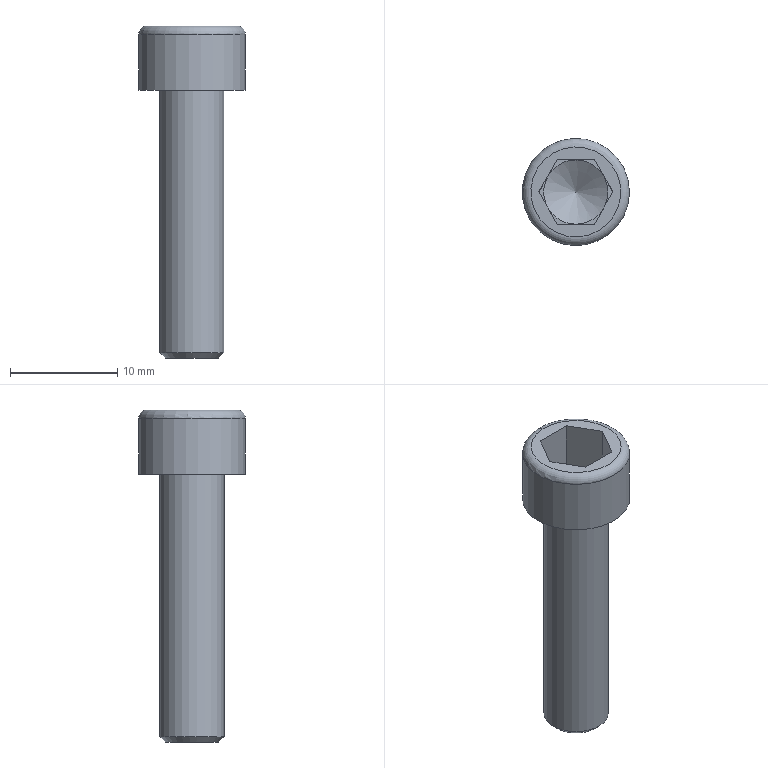Component | NX | GB_T70_1_M6X25_2 | 1 solid | 20 faces | volume 999 mm3 | plane 15 | cylinder 2 | cone 2 | torus 1 | commonest cylinder face diameters 10 x1 6 x1